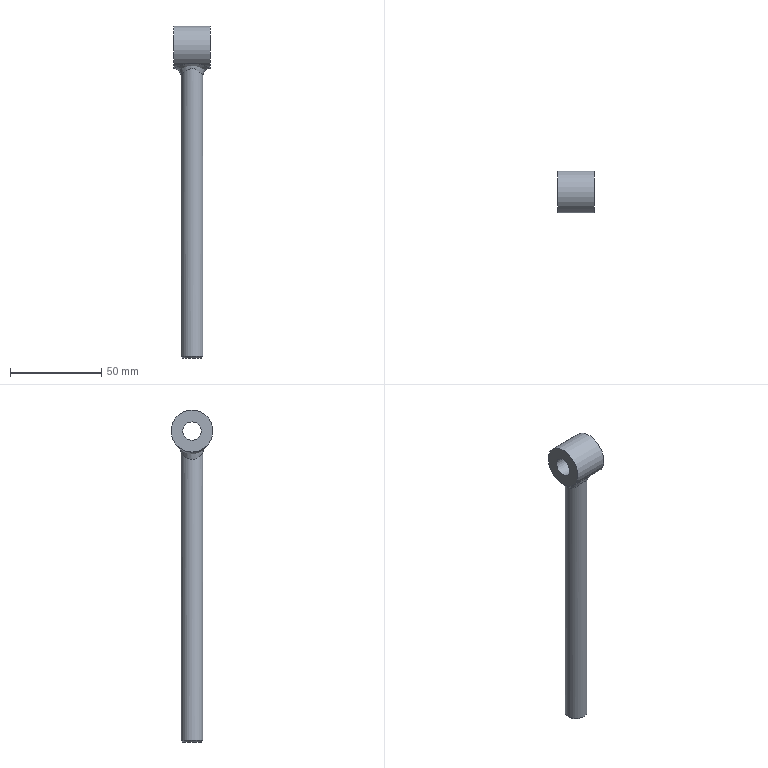Component | NX | SCREW_M12 | 1 solid | 8 faces | volume 24760 mm3 | cylinder 3 | plane 3 | spline 1 | cone 1 | commonest cylinder face diameters 23 x1 12 x1 10 x1